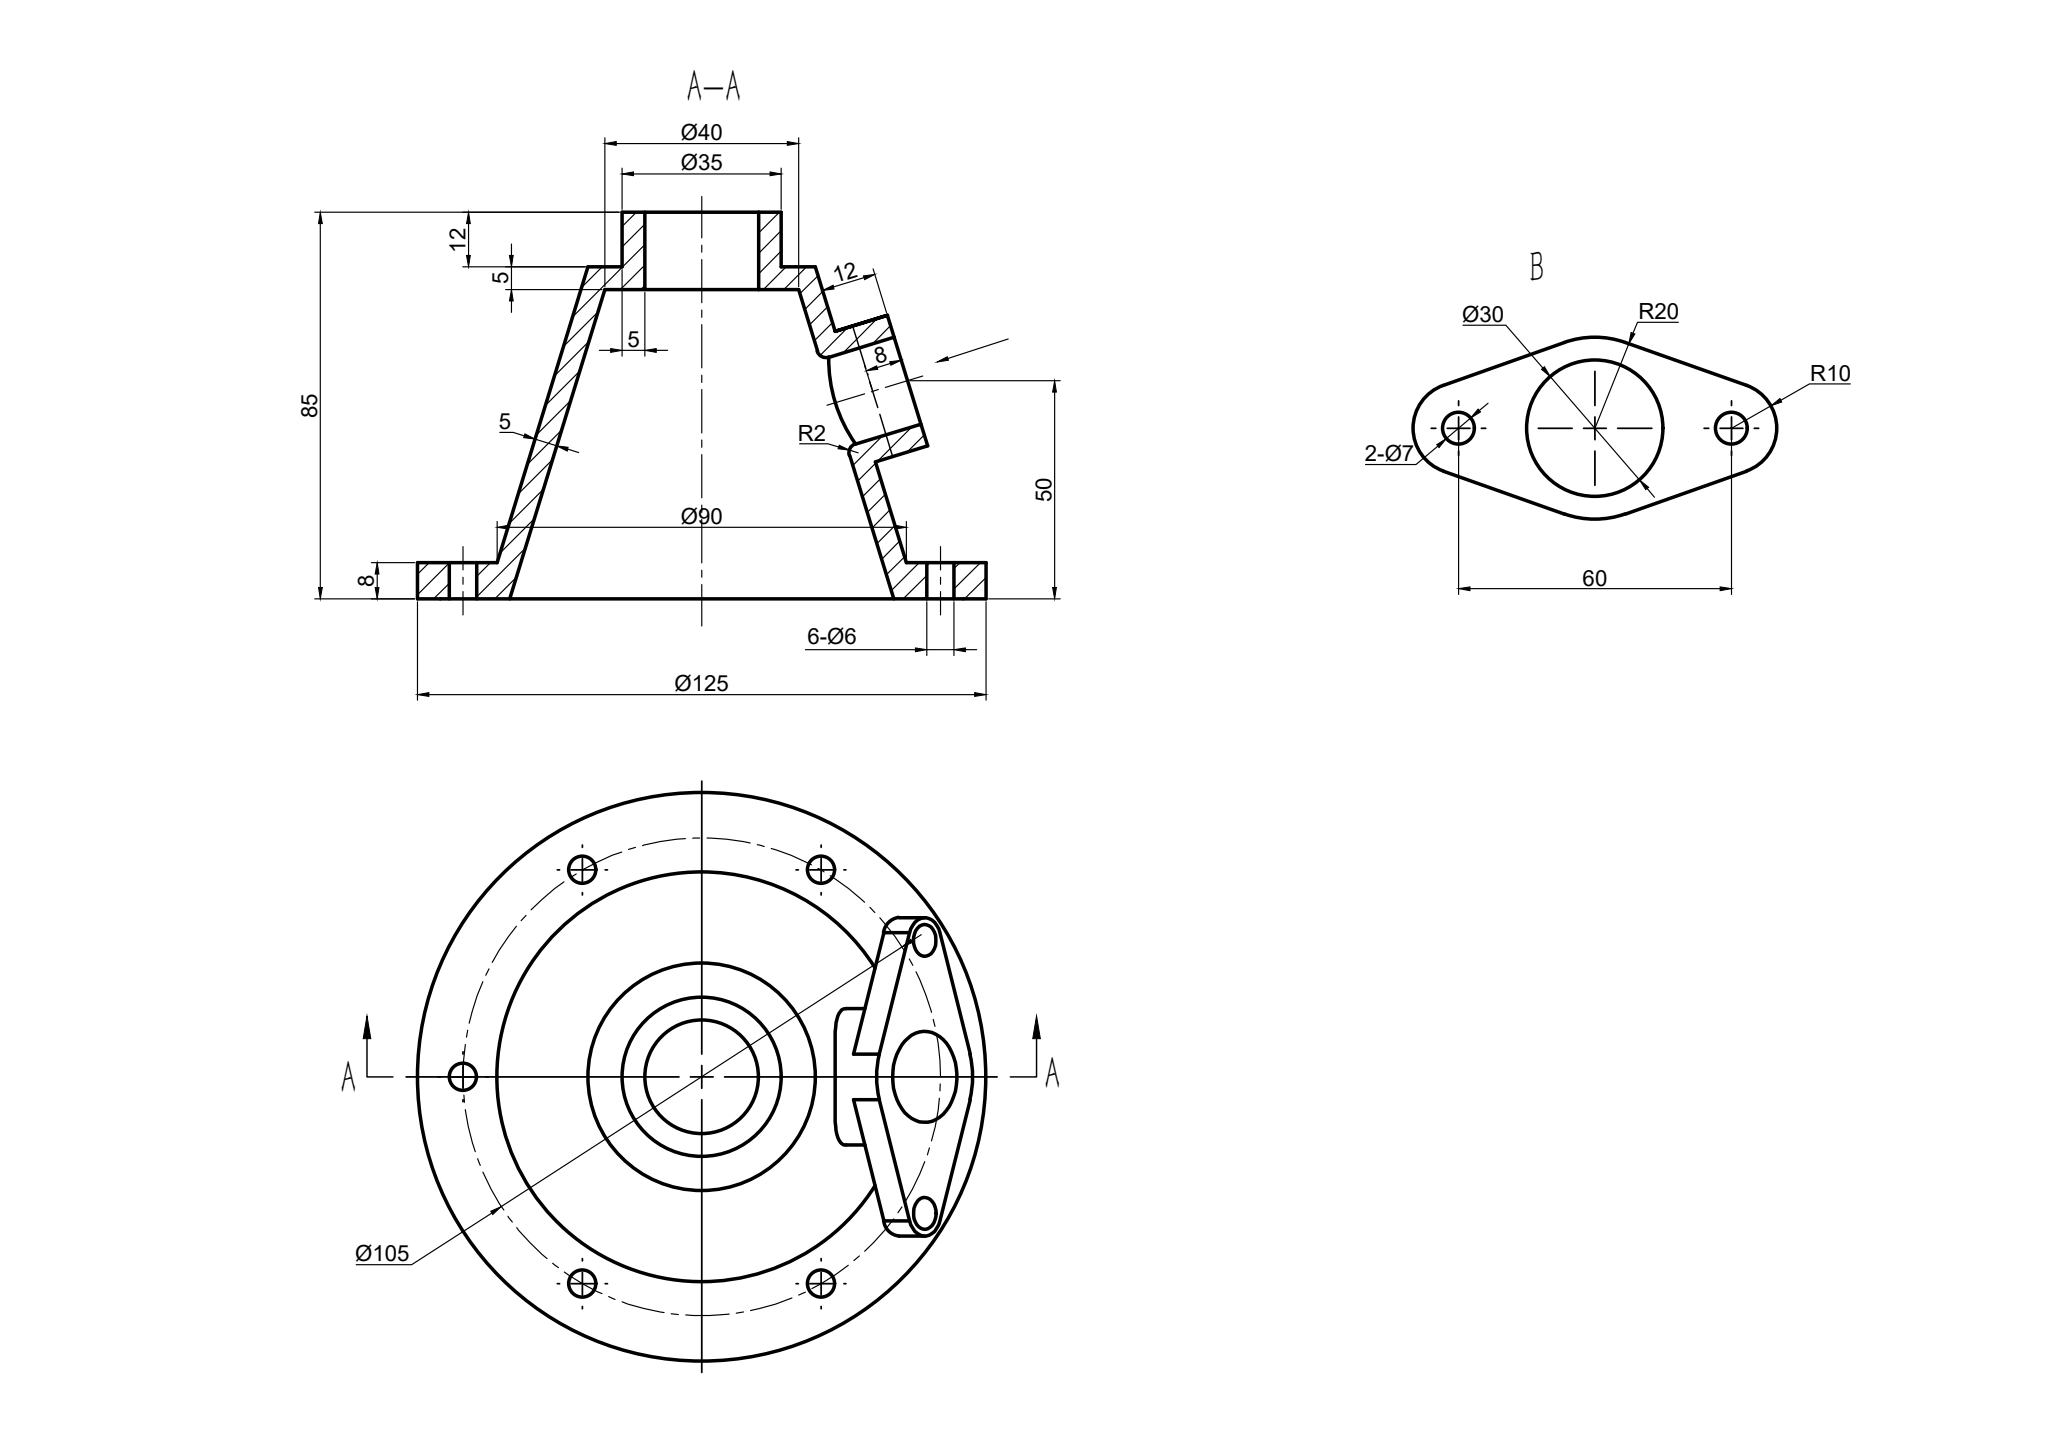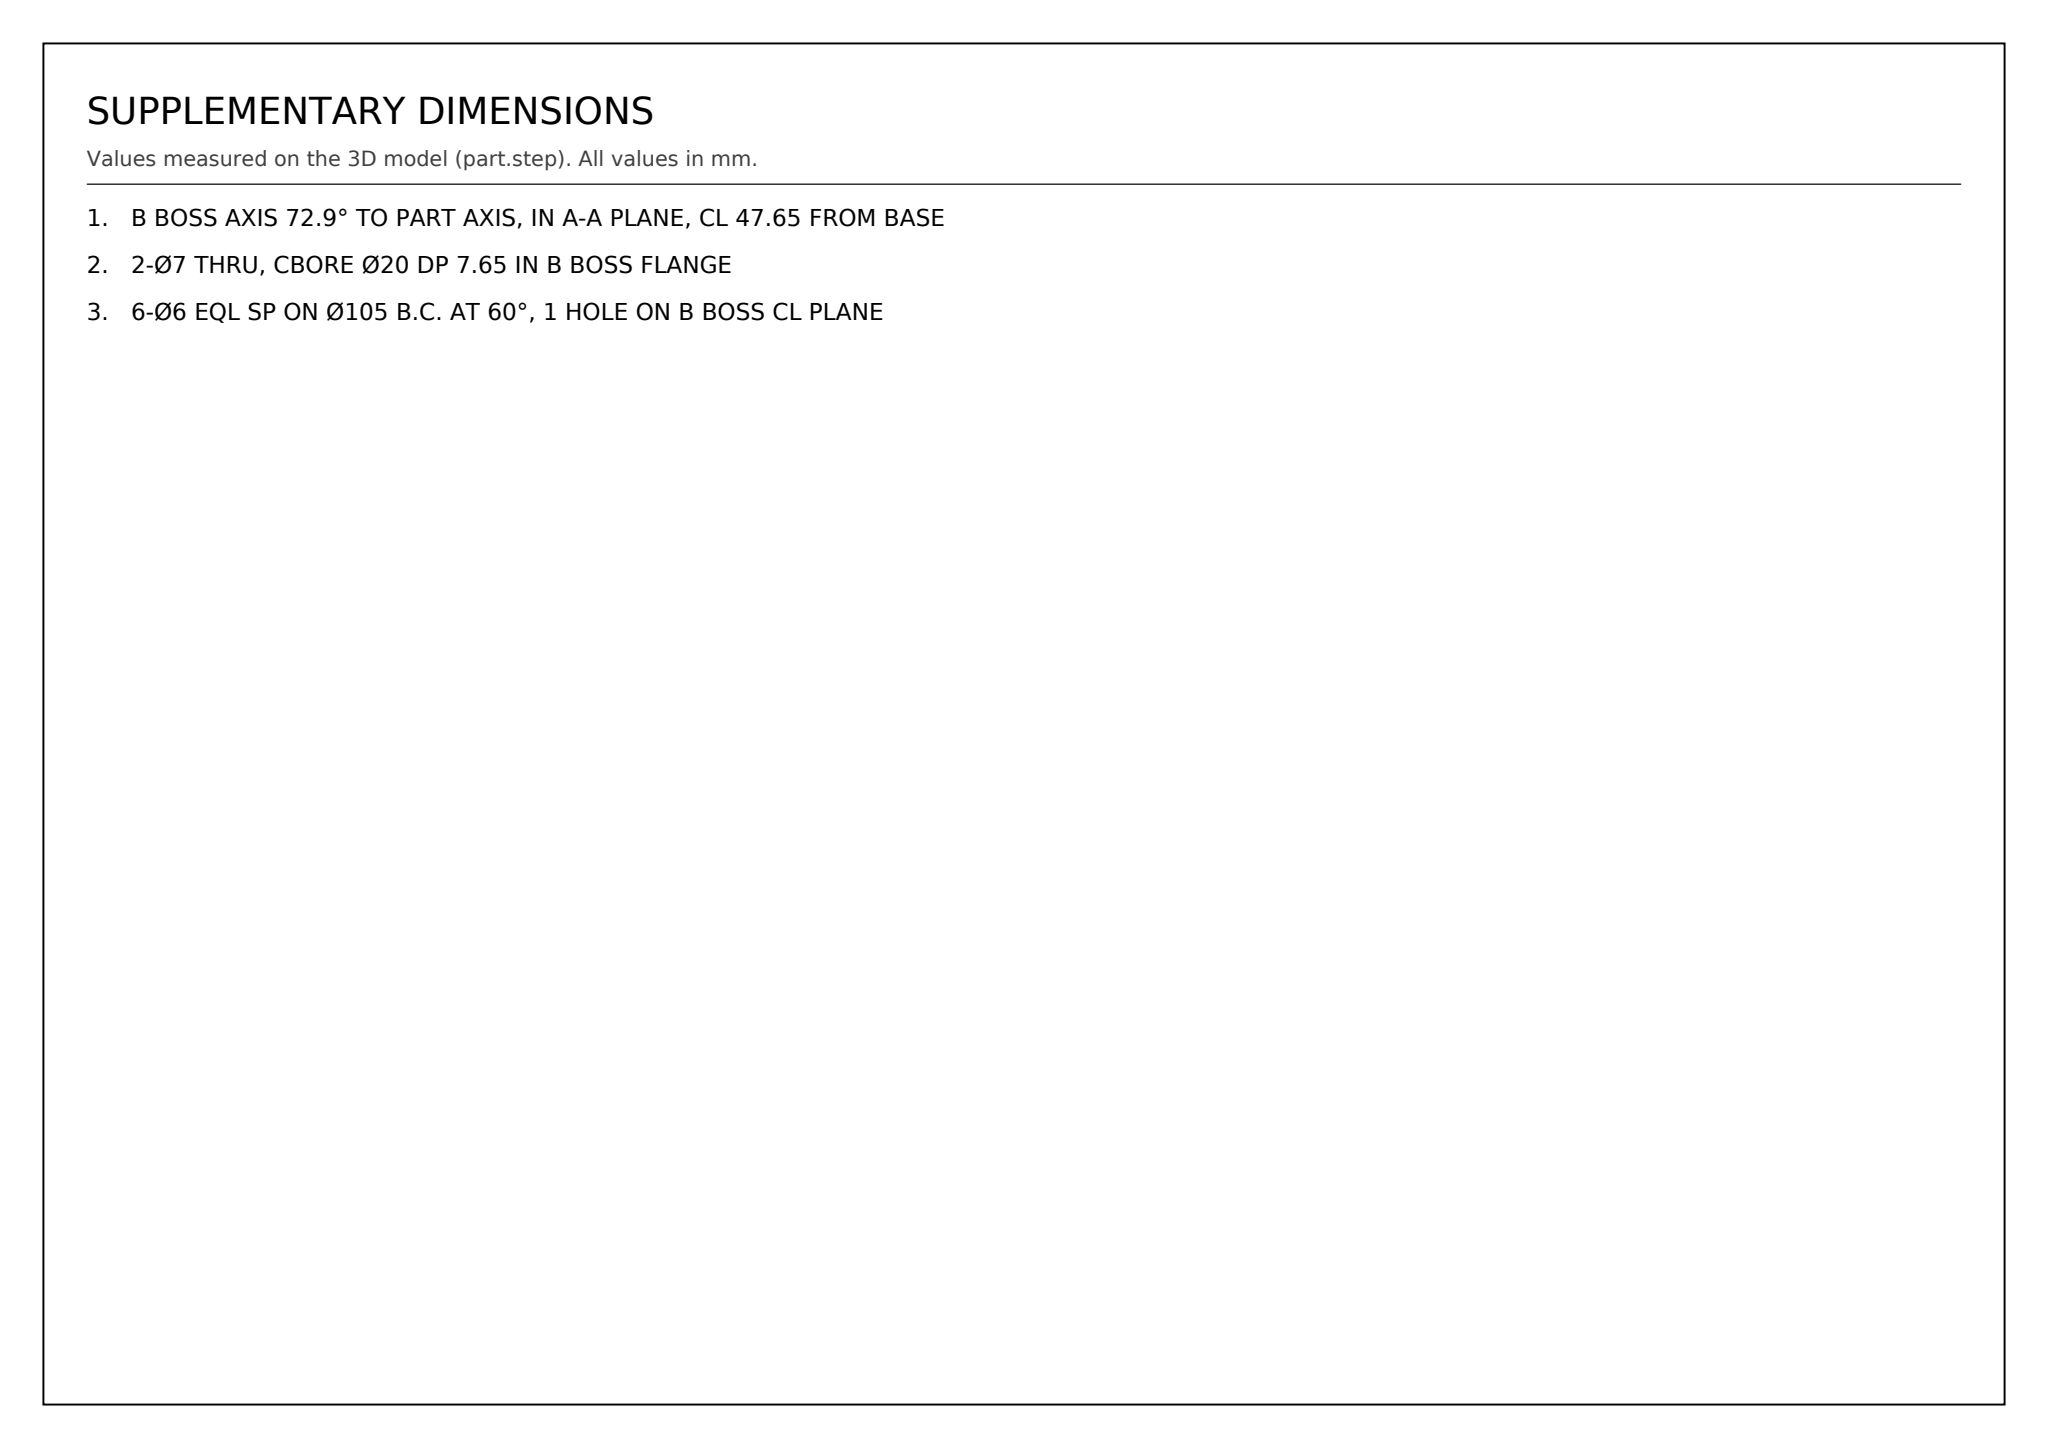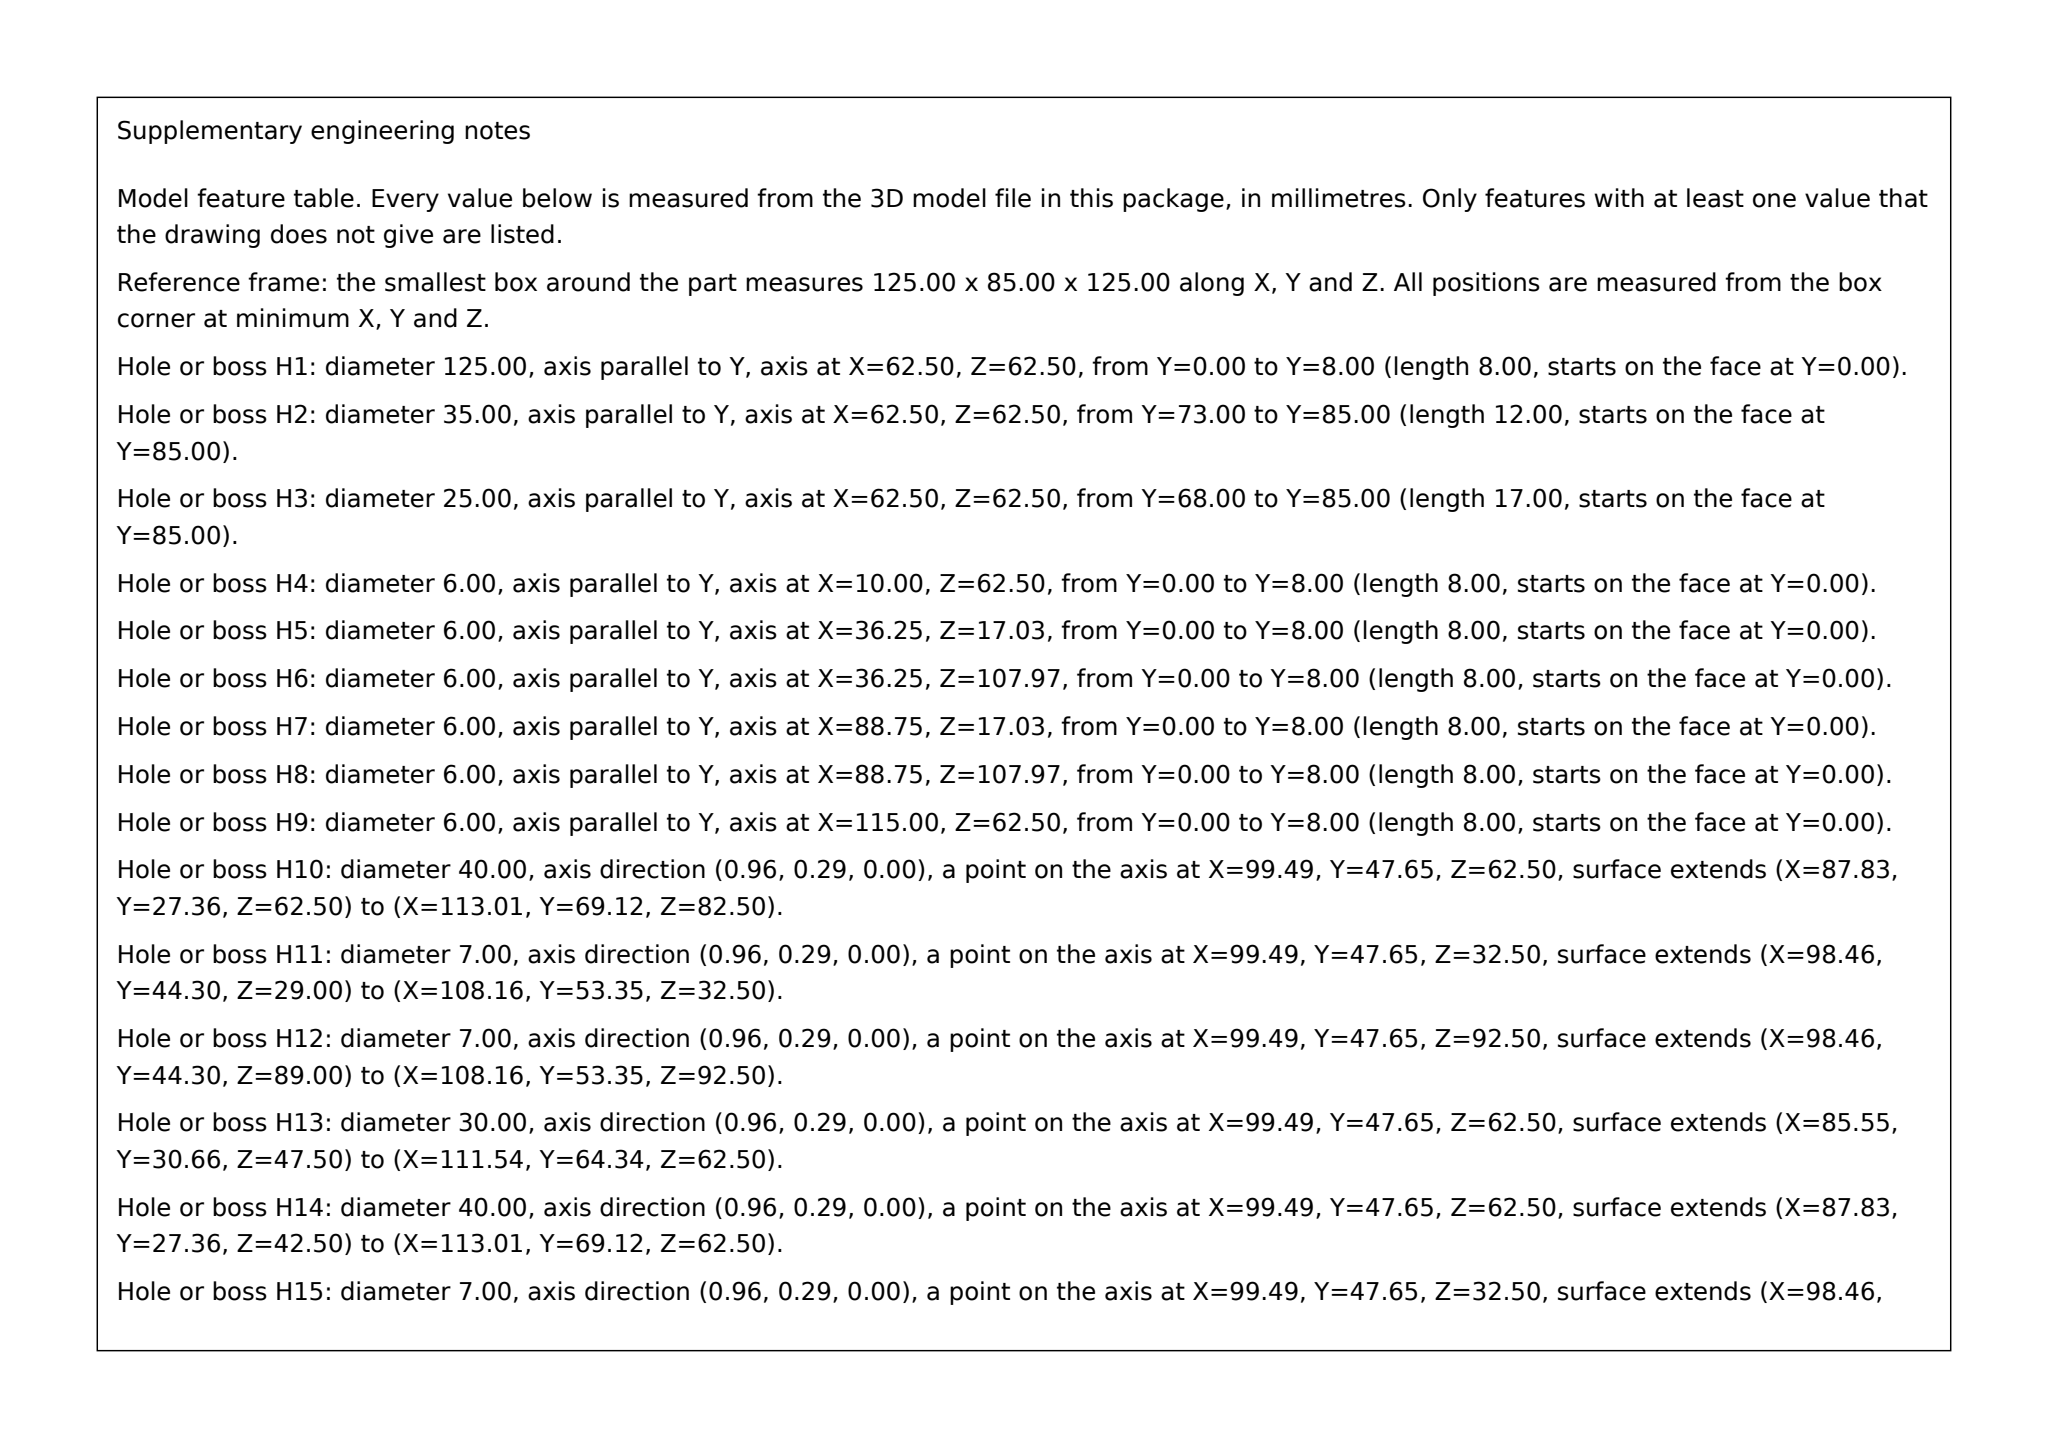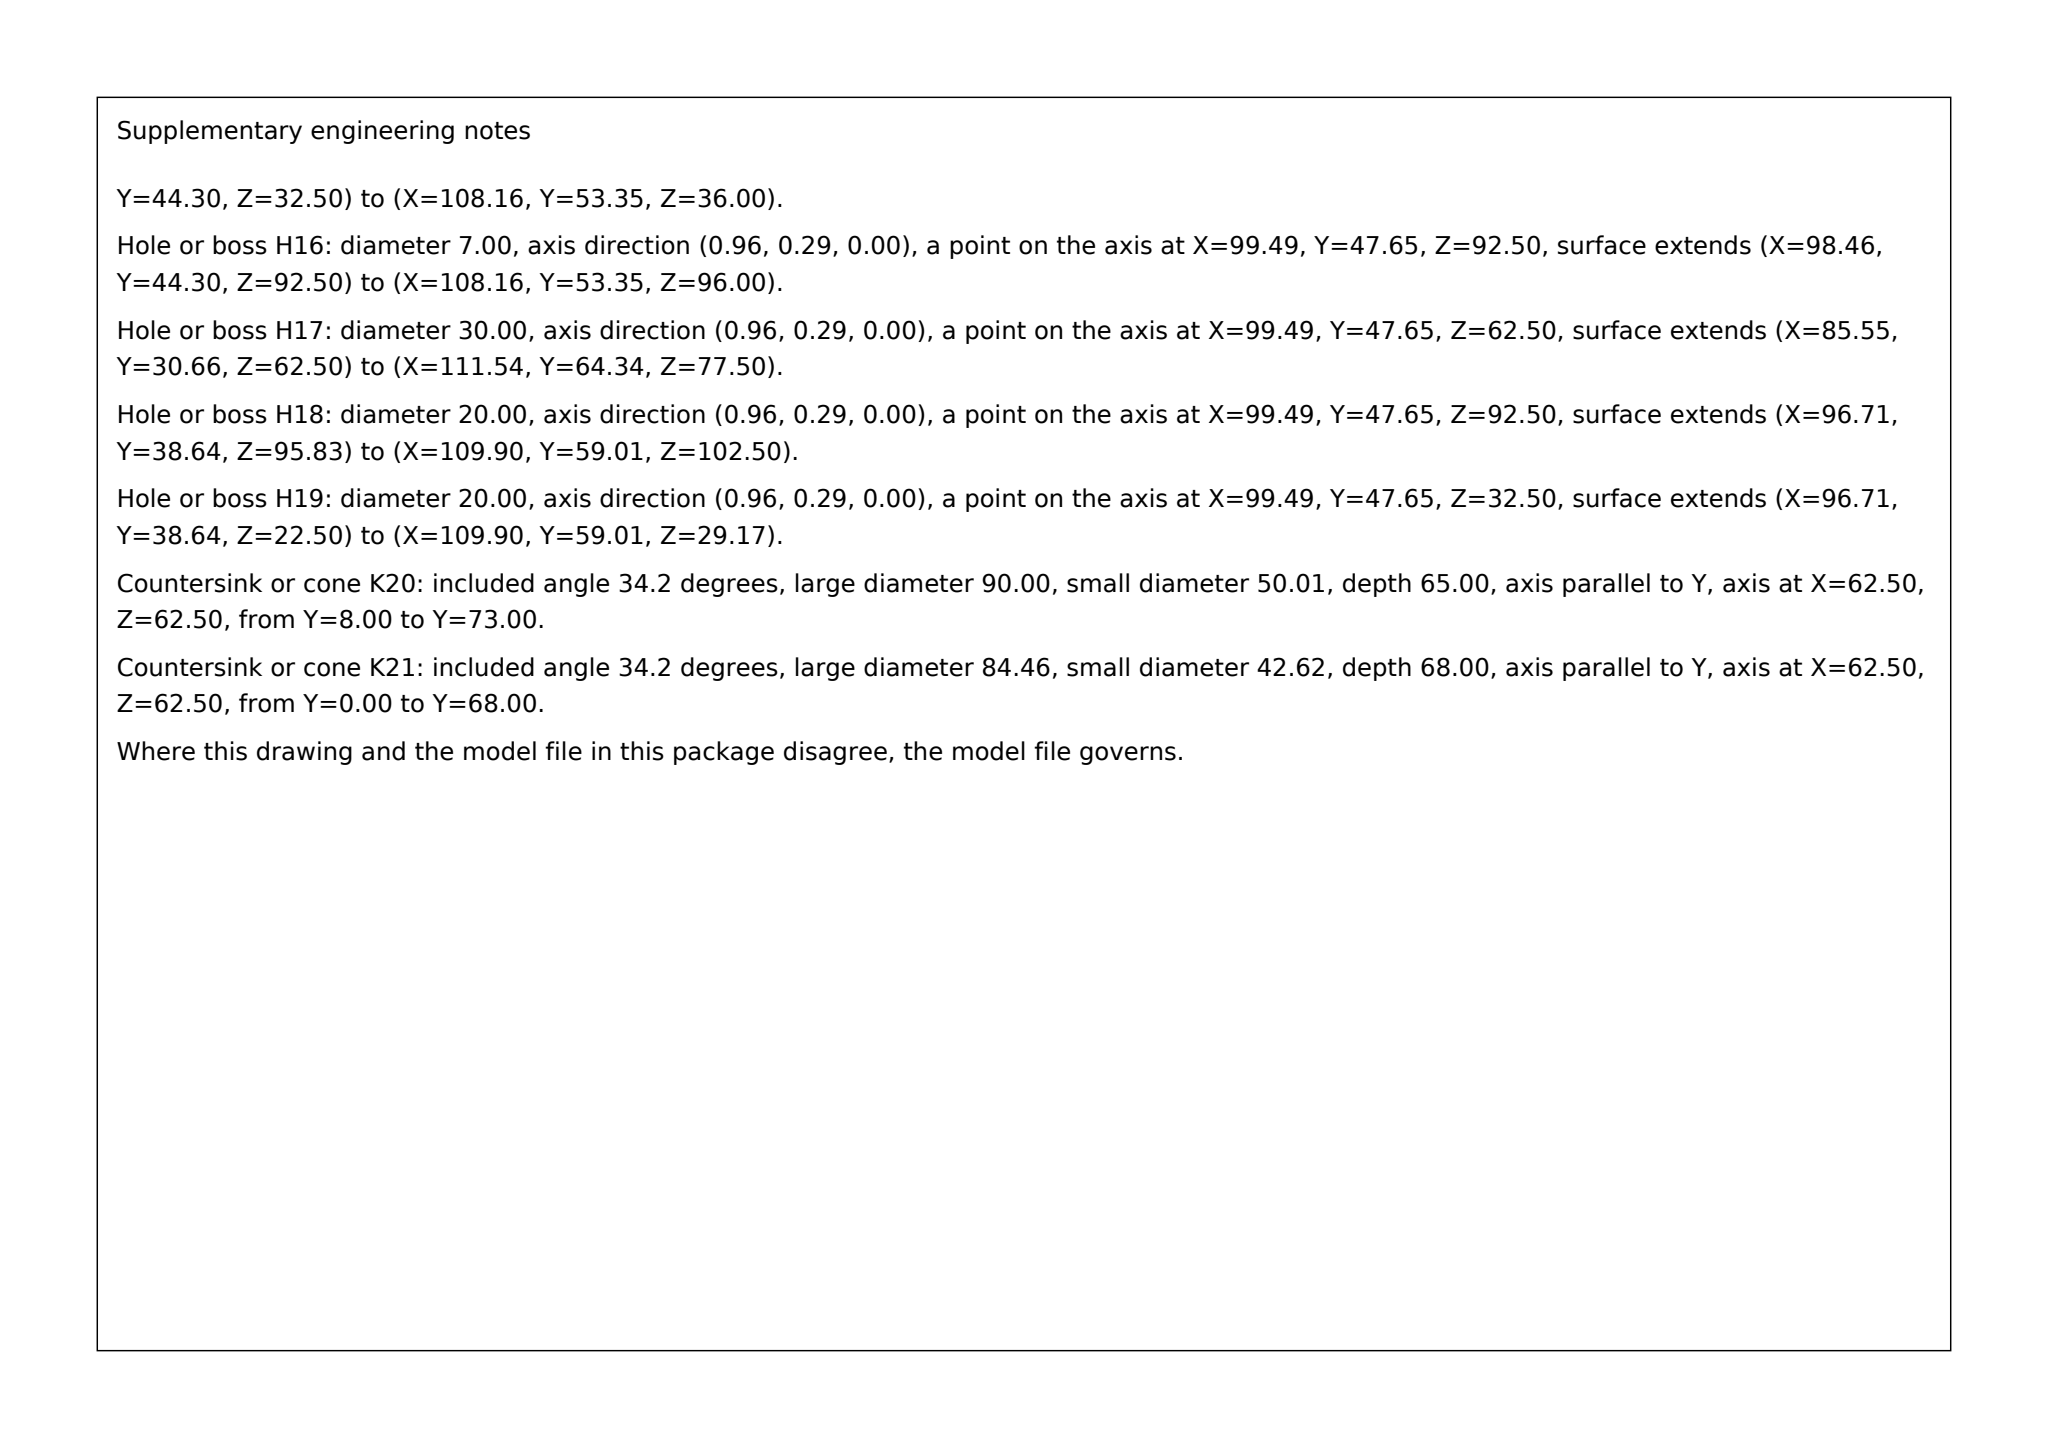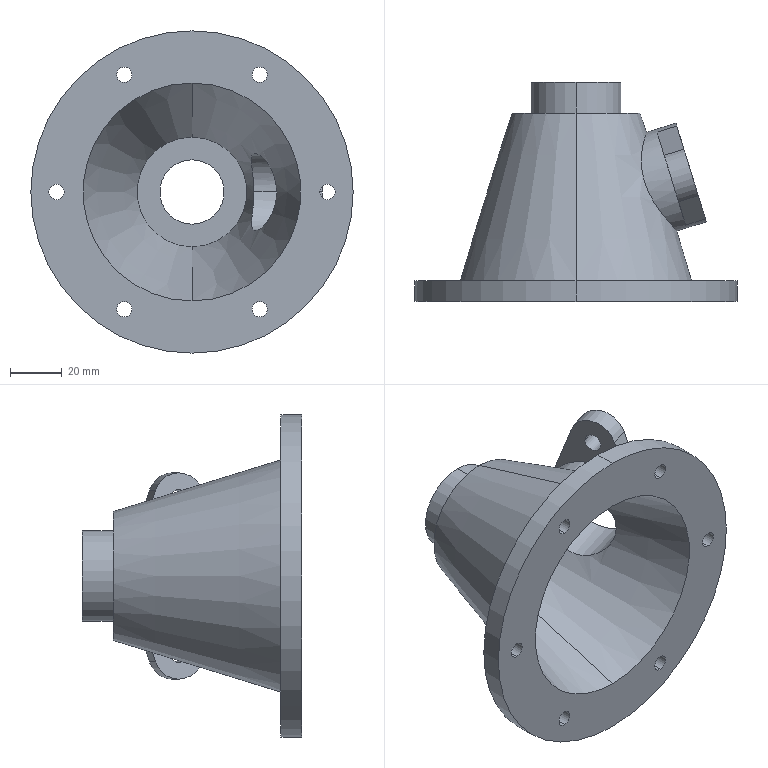Part | SolidWorks | mm | 1 solid | 44 faces | box 125 x 85 x 125 mm | volume 144898 mm3 | cylinder 28 | plane 12 | cone 4 | commonest cylinder face diameters 6 x12 7 x4 125 x2 40 x2 35 x2 30 x2 25 x2 20 x2
Drawing notes:
B BOSS AXIS 72.9° TO PART AXIS, IN A-A PLANE, CL 47.65 FROM BASE | from the solid: cones included angle 34.2 (half 17.1) => boss normal to cone wall = 72.9 deg to vertical axis; boss cyls Ø40/Ø30 axis pos [*,47.65,62.5] = part CL plane z=62.5, 47.65 above bottom face y=0
2-Ø7 THRU, CBORE Ø20 DP 7.65 IN B BOSS FLANGE | from the solid: cylinders [7.0,x,(47.65,32.5/92.5),9.7] and [20.0,x,(47.65,32.5/92.5),13.19]; X-extent 13.19 = L*cos17.1 + 20*sin17.1 -> L=7.65 deep, coaxial with Ø7
6-Ø6 EQL SP ON Ø105 B.C. AT 60°, 1 HOLE ON B BOSS CL PLANE | from the solid: Ø6 y-axis holes at (10,62.5),(36.25,17.03),(36.25,107.97),(88.75,17.03),(88.75,107.97),(115,62.5) about CL (62.5,62.5) = R52.5, 60° spacing, holes at 0° and 180° in A-A/boss plane